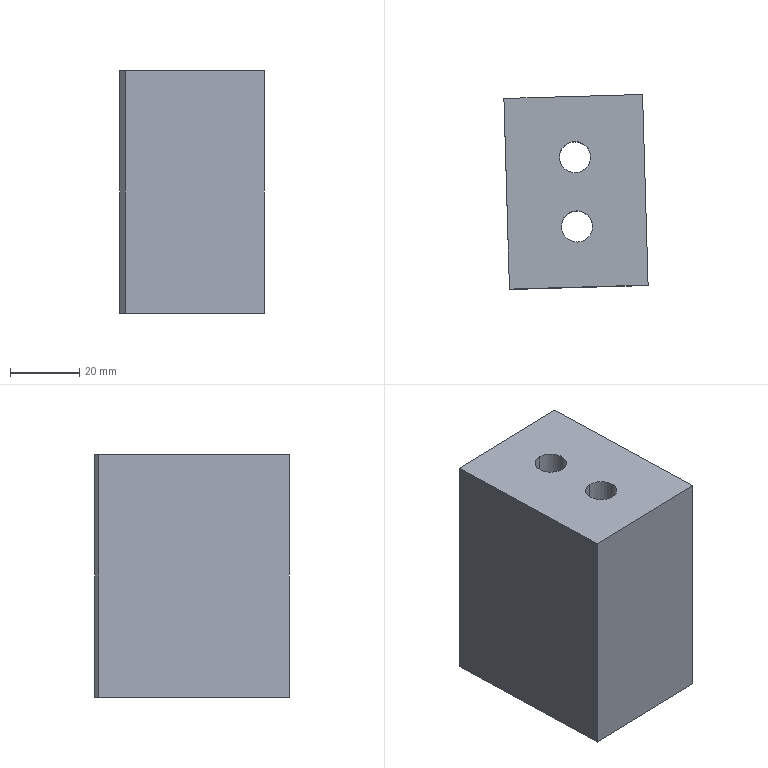Component | SolidWorks | NylonBlock6-1 | 1 solid | 16 faces | box 41.59 x 56.14 x 70 mm | volume 143148 mm3 | cylinder 8 | plane 8 | commonest cylinder face diameters 15 x4 9 x4 | material Nylon 101
build123d program:
from build123d import *

# Parameters (mm, degrees)
SKETCH1_W                                       = 55
SKETCH1_H                                       = 40
BOSS_EXTRUDE1_DEPTH                             = 35
M8_HEX_SOCKET_HEAD_CAP_SCREW_CBORE1_D           = 9
M8_HEX_SOCKET_HEAD_CAP_SCREW_CBORE1_CBORE_D     = 15
M8_HEX_SOCKET_HEAD_CAP_SCREW_CBORE1_CBORE_DEPTH = 8.6


with BuildPart() as part:
    # Sketch1 → Boss-Extrude1 (new, symmetric)
    with BuildSketch(Plane.XY):
        Rectangle(SKETCH1_W, SKETCH1_H)
    extrude(amount=BOSS_EXTRUDE1_DEPTH, both=True)

    # M8 Hex Socket Head Cap Screw CBORE1 (through all)
    with Locations(Plane(origin=(10, 0, -35), x_dir=(-1, 0, 0), z_dir=(0, 0, -1))):
        with Locations((0, 0), (20, 0)):
            CounterBoreHole(M8_HEX_SOCKET_HEAD_CAP_SCREW_CBORE1_D / 2, M8_HEX_SOCKET_HEAD_CAP_SCREW_CBORE1_CBORE_D / 2, M8_HEX_SOCKET_HEAD_CAP_SCREW_CBORE1_CBORE_DEPTH)


solid = part.part

# Placed as in the assembly
solid = solid.moved(Location((-297.687, -220.739, -1261.21), (0, 0, 91.672)))
STEP:
#1=COLOUR_RGB('',0.7922,0.8196,0.9333);
#2=FILL_AREA_STYLE_COLOUR('',#1);
#3=FILL_AREA_STYLE('',(#2));
#4=SURFACE_STYLE_FILL_AREA(#3);
#5=SURFACE_SIDE_STYLE('',(#4));
#6=SURFACE_STYLE_USAGE(.BOTH.,#5);
#7=PRESENTATION_STYLE_ASSIGNMENT((#6));
#8=CARTESIAN_POINT('',(-11.7,-9.379,-50.693));
#9=VERTEX_POINT('',#8);
#10=CARTESIAN_POINT('',(-11.717,-8.789,-50.693));
#11=VERTEX_POINT('',#10);
#12=CARTESIAN_POINT('',(-11.708,-9.084,-50.693));
#13=DIRECTION('',(-0.,0.,-1.));
#14=DIRECTION('',(-0.02918,0.9996,0.));
#15=AXIS2_PLACEMENT_3D('',#12,#13,#14);
#16=CIRCLE('',#15,0.2953);
#17=EDGE_CURVE('',#9,#11,#16,.T.);
#18=ORIENTED_EDGE('',*,*,#17,.F.);
#19=CARTESIAN_POINT('',(-11.7,-9.379,-51.032));
#20=VERTEX_POINT('',#19);
#21=CARTESIAN_POINT('',(-11.7,-9.379,-51.032));
#22=DIRECTION('',(-0.,0.,-1.));
#23=VECTOR('',#22,39.37);
#24=LINE('',#21,#23);
#25=EDGE_CURVE('',#9,#20,#24,.T.);
#26=ORIENTED_EDGE('',*,*,#25,.T.);
#27=CARTESIAN_POINT('',(-11.717,-8.789,-51.032));
#28=VERTEX_POINT('',#27);
#29=CARTESIAN_POINT('',(-11.708,-9.084,-51.032));
#30=DIRECTION('',(-0.,0.,-1.));
#31=DIRECTION('',(-0.02918,0.9996,0.));
#32=AXIS2_PLACEMENT_3D('',#29,#30,#31);
#33=CIRCLE('',#32,0.2953);
#34=EDGE_CURVE('',#20,#28,#33,.T.);
#35=ORIENTED_EDGE('',*,*,#34,.T.);
#36=CARTESIAN_POINT('',(-11.717,-8.789,-51.032));
#37=DIRECTION('',(-0.,0.,-1.));
#38=VECTOR('',#37,39.37);
#39=LINE('',#36,#38);
#40=EDGE_CURVE('',#11,#28,#39,.T.);
#41=ORIENTED_EDGE('',*,*,#40,.F.);
#42=EDGE_LOOP('',(#18,#26,#35,#41));
#43=FACE_OUTER_BOUND('',#42,.T.);
#44=CARTESIAN_POINT('',(-11.708,-9.084,-51.032));
#45=DIRECTION('',(-0.,0.,-1.));
#46=DIRECTION('',(-0.02918,0.9996,0.));
#47=AXIS2_PLACEMENT_3D('',#44,#45,#46);
#48=CYLINDRICAL_SURFACE('',#47,0.2953);
#49=ADVANCED_FACE('',(#43),#48,.F.);
#50=CARTESIAN_POINT('',(-11.703,-9.261,-48.276));
#51=VERTEX_POINT('',#50);
#52=CARTESIAN_POINT('',(-11.714,-8.907,-48.276));
#53=VERTEX_POINT('',#52);
#54=CARTESIAN_POINT('',(-11.708,-9.084,-48.276));
#55=DIRECTION('',(-0.,0.,-1.));
#56=DIRECTION('',(-0.02918,0.9996,0.));
#57=AXIS2_PLACEMENT_3D('',#54,#55,#56);
#58=CIRCLE('',#57,0.1772);
#59=EDGE_CURVE('',#51,#53,#58,.T.);
#60=ORIENTED_EDGE('',*,*,#59,.F.);
#61=CARTESIAN_POINT('',(-11.703,-9.261,-50.693));
#62=VERTEX_POINT('',#61);
#63=CARTESIAN_POINT('',(-11.703,-9.261,-51.032));
#64=DIRECTION('',(-0.,0.,-1.));
#65=VECTOR('',#64,39.37);
#66=LINE('',#63,#65);
#67=EDGE_CURVE('',#51,#62,#66,.T.);
#68=ORIENTED_EDGE('',*,*,#67,.T.);
#69=CARTESIAN_POINT('',(-11.714,-8.907,-50.693));
#70=VERTEX_POINT('',#69);
#71=CARTESIAN_POINT('',(-11.708,-9.084,-50.693));
#72=DIRECTION('',(-0.,0.,-1.));
#73=DIRECTION('',(-0.02918,0.9996,0.));
#74=AXIS2_PLACEMENT_3D('',#71,#72,#73);
#75=CIRCLE('',#74,0.1772);
#76=EDGE_CURVE('',#62,#70,#75,.T.);
#77=ORIENTED_EDGE('',*,*,#76,.T.);
#78=CARTESIAN_POINT('',(-11.714,-8.907,-51.032));
#79=DIRECTION('',(-0.,0.,-1.));
#80=VECTOR('',#79,39.37);
#81=LINE('',#78,#80);
#82=EDGE_CURVE('',#53,#70,#81,.T.);
#83=ORIENTED_EDGE('',*,*,#82,.F.);
#84=EDGE_LOOP('',(#60,#68,#77,#83));
#85=FACE_OUTER_BOUND('',#84,.T.);
#86=CARTESIAN_POINT('',(-11.708,-9.084,-51.032));
#87=DIRECTION('',(-0.,0.,-1.));
#88=DIRECTION('',(-0.02918,0.9996,0.));
#89=AXIS2_PLACEMENT_3D('',#86,#87,#88);
#90=CYLINDRICAL_SURFACE('',#89,0.1772);
#91=ADVANCED_FACE('',(#85),#90,.F.);
#92=CARTESIAN_POINT('',(-11.723,-8.592,-50.693));
#93=VERTEX_POINT('',#92);
#94=CARTESIAN_POINT('',(-11.74,-8.002,-50.693));
#95=VERTEX_POINT('',#94);
#96=CARTESIAN_POINT('',(-11.731,-8.297,-50.693));
#97=DIRECTION('',(-0.,0.,-1.));
#98=DIRECTION('',(-0.02918,0.9996,0.));
#99=AXIS2_PLACEMENT_3D('',#96,#97,#98);
#100=CIRCLE('',#99,0.2953);
#101=EDGE_CURVE('',#93,#95,#100,.T.);
#102=ORIENTED_EDGE('',*,*,#101,.F.);
#103=CARTESIAN_POINT('',(-11.723,-8.592,-51.032));
#104=VERTEX_POINT('',#103);
#105=CARTESIAN_POINT('',(-11.723,-8.592,-51.032));
#106=DIRECTION('',(-0.,0.,-1.));
#107=VECTOR('',#106,39.37);
#108=LINE('',#105,#107);
#109=EDGE_CURVE('',#93,#104,#108,.T.);
#110=ORIENTED_EDGE('',*,*,#109,.T.);
#111=CARTESIAN_POINT('',(-11.74,-8.002,-51.032));
#112=VERTEX_POINT('',#111);
#113=CARTESIAN_POINT('',(-11.731,-8.297,-51.032));
#114=DIRECTION('',(-0.,0.,-1.));
#115=DIRECTION('',(-0.02918,0.9996,0.));
#116=AXIS2_PLACEMENT_3D('',#113,#114,#115);
#117=CIRCLE('',#116,0.2953);
#118=EDGE_CURVE('',#104,#112,#117,.T.);
#119=ORIENTED_EDGE('',*,*,#118,.T.);
#120=CARTESIAN_POINT('',(-11.74,-8.002,-51.032));
#121=DIRECTION('',(-0.,0.,-1.));
#122=VECTOR('',#121,39.37);
#123=LINE('',#120,#122);
#124=EDGE_CURVE('',#95,#112,#123,.T.);
#125=ORIENTED_EDGE('',*,*,#124,.F.);
#126=EDGE_LOOP('',(#102,#110,#119,#125));
#127=FACE_OUTER_BOUND('',#126,.T.);
#128=CARTESIAN_POINT('',(-11.731,-8.297,-51.032));
#129=DIRECTION('',(-0.,0.,-1.));
#130=DIRECTION('',(-0.02918,0.9996,0.));
#131=AXIS2_PLACEMENT_3D('',#128,#129,#130);
#132=CYLINDRICAL_SURFACE('',#131,0.2953);
#133=ADVANCED_FACE('',(#127),#132,.F.);
#134=CARTESIAN_POINT('',(-11.726,-8.474,-48.276));
#135=VERTEX_POINT('',#134);
#136=CARTESIAN_POINT('',(-11.737,-8.12,-48.276));
#137=VERTEX_POINT('',#136);
#138=CARTESIAN_POINT('',(-11.731,-8.297,-48.276));
#139=DIRECTION('',(-0.,0.,-1.));
#140=DIRECTION('',(-0.02918,0.9996,0.));
#141=AXIS2_PLACEMENT_3D('',#138,#139,#140);
#142=CIRCLE('',#141,0.1772);
#143=EDGE_CURVE('',#135,#137,#142,.T.);
#144=ORIENTED_EDGE('',*,*,#143,.F.);
#145=CARTESIAN_POINT('',(-11.726,-8.474,-50.693));
#146=VERTEX_POINT('',#145);
#147=CARTESIAN_POINT('',(-11.726,-8.474,-51.032));
#148=DIRECTION('',(-0.,0.,-1.));
#149=VECTOR('',#148,39.37);
#150=LINE('',#147,#149);
#151=EDGE_CURVE('',#135,#146,#150,.T.);
#152=ORIENTED_EDGE('',*,*,#151,.T.);
#153=CARTESIAN_POINT('',(-11.737,-8.12,-50.693));
#154=VERTEX_POINT('',#153);
#155=CARTESIAN_POINT('',(-11.731,-8.297,-50.693));
#156=DIRECTION('',(-0.,0.,-1.));
#157=DIRECTION('',(-0.02918,0.9996,0.));
#158=AXIS2_PLACEMENT_3D('',#155,#156,#157);
#159=CIRCLE('',#158,0.1772);
#160=EDGE_CURVE('',#146,#154,#159,.T.);
#161=ORIENTED_EDGE('',*,*,#160,.T.);
#162=CARTESIAN_POINT('',(-11.737,-8.12,-51.032));
#163=DIRECTION('',(-0.,0.,-1.));
#164=VECTOR('',#163,39.37);
#165=LINE('',#162,#164);
#166=EDGE_CURVE('',#137,#154,#165,.T.);
#167=ORIENTED_EDGE('',*,*,#166,.F.);
#168=EDGE_LOOP('',(#144,#152,#161,#167));
#169=FACE_OUTER_BOUND('',#168,.T.);
#170=CARTESIAN_POINT('',(-11.731,-8.297,-51.032));
#171=DIRECTION('',(-0.,0.,-1.));
#172=DIRECTION('',(-0.02918,0.9996,0.));
#173=AXIS2_PLACEMENT_3D('',#170,#171,#172);
#174=CYLINDRICAL_SURFACE('',#173,0.1772);
#175=ADVANCED_FACE('',(#169),#174,.F.);
#176=CARTESIAN_POINT('',(-12.475,-9.796,-51.032));
#177=VERTEX_POINT('',#176);
#178=CARTESIAN_POINT('',(-10.901,-9.75,-51.032));
#179=VERTEX_POINT('',#178);
#180=CARTESIAN_POINT('',(-10.901,-9.75,-51.032));
#181=DIRECTION('',(0.9996,0.02918,-0.));
#182=VECTOR('',#181,39.37);
#183=LINE('',#180,#182);
#184=EDGE_CURVE('',#177,#179,#183,.T.);
#185=ORIENTED_EDGE('',*,*,#184,.T.);
#186=CARTESIAN_POINT('',(-10.901,-9.75,-48.276));
#187=VERTEX_POINT('',#186);
#188=CARTESIAN_POINT('',(-10.901,-9.75,-48.276));
#189=DIRECTION('',(-0.,0.,-1.));
#190=VECTOR('',#189,39.37);
#191=LINE('',#188,#190);
#192=EDGE_CURVE('',#187,#179,#191,.T.);
#193=ORIENTED_EDGE('',*,*,#192,.F.);
#194=CARTESIAN_POINT('',(-12.475,-9.796,-48.276));
#195=VERTEX_POINT('',#194);
#196=CARTESIAN_POINT('',(-10.901,-9.75,-48.276));
#197=DIRECTION('',(0.9996,0.02918,-0.));
#198=VECTOR('',#197,39.37);
#199=LINE('',#196,#198);
#200=EDGE_CURVE('',#195,#187,#199,.T.);
#201=ORIENTED_EDGE('',*,*,#200,.F.);
#202=CARTESIAN_POINT('',(-12.475,-9.796,-48.276));
#203=DIRECTION('',(-0.,0.,-1.));
#204=VECTOR('',#203,39.37);
#205=LINE('',#202,#204);
#206=EDGE_CURVE('',#195,#177,#205,.T.);
#207=ORIENTED_EDGE('',*,*,#206,.T.);
#208=EDGE_LOOP('',(#185,#193,#201,#207));
#209=FACE_OUTER_BOUND('',#208,.T.);
#210=CARTESIAN_POINT('',(-10.901,-9.75,-48.276));
#211=DIRECTION('',(-0.02918,0.9996,0.));
#212=DIRECTION('',(-0.9996,-0.02918,0.));
#213=AXIS2_PLACEMENT_3D('',#210,#211,#212);
#214=PLANE('',#213);
#215=ADVANCED_FACE('',(#209),#214,.F.);
#216=CARTESIAN_POINT('',(-10.964,-7.585,-51.032));
#217=VERTEX_POINT('',#216);
#218=CARTESIAN_POINT('',(-10.964,-7.585,-51.032));
#219=DIRECTION('',(-0.02918,0.9996,0.));
#220=VECTOR('',#219,39.37);
#221=LINE('',#218,#220);
#222=EDGE_CURVE('',#179,#217,#221,.T.);
#223=ORIENTED_EDGE('',*,*,#222,.T.);
#224=CARTESIAN_POINT('',(-10.964,-7.585,-48.276));
#225=VERTEX_POINT('',#224);
#226=CARTESIAN_POINT('',(-10.964,-7.585,-48.276));
#227=DIRECTION('',(-0.,0.,-1.));
#228=VECTOR('',#227,39.37);
#229=LINE('',#226,#228);
#230=EDGE_CURVE('',#225,#217,#229,.T.);
#231=ORIENTED_EDGE('',*,*,#230,.F.);
#232=CARTESIAN_POINT('',(-10.964,-7.585,-48.276));
#233=DIRECTION('',(-0.02918,0.9996,0.));
#234=VECTOR('',#233,39.37);
#235=LINE('',#232,#234);
#236=EDGE_CURVE('',#187,#225,#235,.T.);
#237=ORIENTED_EDGE('',*,*,#236,.F.);
#238=ORIENTED_EDGE('',*,*,#192,.T.);
#239=EDGE_LOOP('',(#223,#231,#237,#238));
#240=FACE_OUTER_BOUND('',#239,.T.);
#241=CARTESIAN_POINT('',(-10.964,-7.585,-48.276));
#242=DIRECTION('',(-0.9996,-0.02918,0.));
#243=DIRECTION('',(-0.,0.,-1.));
#244=AXIS2_PLACEMENT_3D('',#241,#242,#243);
#245=PLANE('',#244);
#246=ADVANCED_FACE('',(#240),#245,.F.);
#247=CARTESIAN_POINT('',(-12.539,-7.631,-51.032));
#248=VERTEX_POINT('',#247);
#249=CARTESIAN_POINT('',(-10.964,-7.585,-51.032));
#250=DIRECTION('',(-0.9996,-0.02918,0.));
#251=VECTOR('',#250,39.37);
#252=LINE('',#249,#251);
#253=EDGE_CURVE('',#217,#248,#252,.T.);
#254=ORIENTED_EDGE('',*,*,#253,.T.);
#255=CARTESIAN_POINT('',(-12.539,-7.631,-48.276));
#256=VERTEX_POINT('',#255);
#257=CARTESIAN_POINT('',(-12.539,-7.631,-48.276));
#258=DIRECTION('',(-0.,0.,-1.));
#259=VECTOR('',#258,39.37);
#260=LINE('',#257,#259);
#261=EDGE_CURVE('',#256,#248,#260,.T.);
#262=ORIENTED_EDGE('',*,*,#261,.F.);
#263=CARTESIAN_POINT('',(-10.964,-7.585,-48.276));
#264=DIRECTION('',(-0.9996,-0.02918,0.));
#265=VECTOR('',#264,39.37);
#266=LINE('',#263,#265);
#267=EDGE_CURVE('',#225,#256,#266,.T.);
#268=ORIENTED_EDGE('',*,*,#267,.F.);
#269=ORIENTED_EDGE('',*,*,#230,.T.);
#270=EDGE_LOOP('',(#254,#262,#268,#269));
#271=FACE_OUTER_BOUND('',#270,.T.);
#272=CARTESIAN_POINT('',(-10.964,-7.585,-48.276));
#273=DIRECTION('',(0.02918,-0.9996,-0.));
#274=DIRECTION('',(0.9996,0.02918,-0.));
#275=AXIS2_PLACEMENT_3D('',#272,#273,#274);
#276=PLANE('',#275);
#277=ADVANCED_FACE('',(#271),#276,.F.);
#278=CARTESIAN_POINT('',(-12.539,-7.631,-51.032));
#279=DIRECTION('',(0.02918,-0.9996,-0.));
#280=VECTOR('',#279,39.37);
#281=LINE('',#278,#280);
#282=EDGE_CURVE('',#248,#177,#281,.T.);
#283=ORIENTED_EDGE('',*,*,#282,.T.);
#284=ORIENTED_EDGE('',*,*,#206,.F.);
#285=CARTESIAN_POINT('',(-12.539,-7.631,-48.276));
#286=DIRECTION('',(0.02918,-0.9996,-0.));
#287=VECTOR('',#286,39.37);
#288=LINE('',#285,#287);
#289=EDGE_CURVE('',#256,#195,#288,.T.);
#290=ORIENTED_EDGE('',*,*,#289,.F.);
#291=ORIENTED_EDGE('',*,*,#261,.T.);
#292=EDGE_LOOP('',(#283,#284,#290,#291));
#293=FACE_OUTER_BOUND('',#292,.T.);
#294=CARTESIAN_POINT('',(-12.539,-7.631,-48.276));
#295=DIRECTION('',(0.9996,0.02918,-0.));
#296=DIRECTION('',(0.,-0.,1.));
#297=AXIS2_PLACEMENT_3D('',#294,#295,#296);
#298=PLANE('',#297);
#299=ADVANCED_FACE('',(#293),#298,.F.);
#300=CARTESIAN_POINT('',(-11.708,-9.084,-48.276));
#301=DIRECTION('',(-0.,0.,-1.));
#302=DIRECTION('',(-0.02918,0.9996,0.));
#303=AXIS2_PLACEMENT_3D('',#300,#301,#302);
#304=CIRCLE('',#303,0.1772);
#305=EDGE_CURVE('',#53,#51,#304,.T.);
#306=ORIENTED_EDGE('',*,*,#305,.T.);
#307=ORIENTED_EDGE('',*,*,#59,.T.);
#308=EDGE_LOOP('',(#306,#307));
#309=FACE_BOUND('',#308,.T.);
#310=CARTESIAN_POINT('',(-11.731,-8.297,-48.276));
#311=DIRECTION('',(-0.,0.,-1.));
#312=DIRECTION('',(-0.02918,0.9996,0.));
#313=AXIS2_PLACEMENT_3D('',#310,#311,#312);
#314=CIRCLE('',#313,0.1772);
#315=EDGE_CURVE('',#137,#135,#314,.T.);
#316=ORIENTED_EDGE('',*,*,#315,.T.);
#317=ORIENTED_EDGE('',*,*,#143,.T.);
#318=EDGE_LOOP('',(#316,#317));
#319=FACE_BOUND('',#318,.T.);
#320=ORIENTED_EDGE('',*,*,#200,.T.);
#321=ORIENTED_EDGE('',*,*,#236,.T.);
#322=ORIENTED_EDGE('',*,*,#267,.T.);
#323=ORIENTED_EDGE('',*,*,#289,.T.);
#324=EDGE_LOOP('',(#320,#321,#322,#323));
#325=FACE_OUTER_BOUND('',#324,.T.);
#326=CARTESIAN_POINT('',(-11.72,-8.691,-48.276));
#327=DIRECTION('',(0.,-0.,1.));
#328=DIRECTION('',(0.02918,-0.9996,-0.));
#329=AXIS2_PLACEMENT_3D('',#326,#327,#328);
#330=PLANE('',#329);
#331=ADVANCED_FACE('',(#309,#319,#325),#330,.T.);
#332=CARTESIAN_POINT('',(-11.708,-9.084,-51.032));
#333=DIRECTION('',(-0.,0.,-1.));
#334=DIRECTION('',(-0.02918,0.9996,0.));
#335=AXIS2_PLACEMENT_3D('',#332,#333,#334);
#336=CIRCLE('',#335,0.2953);
#337=EDGE_CURVE('',#28,#20,#336,.T.);
#338=ORIENTED_EDGE('',*,*,#337,.F.);
#339=ORIENTED_EDGE('',*,*,#34,.F.);
#340=EDGE_LOOP('',(#338,#339));
#341=FACE_BOUND('',#340,.T.);
#342=CARTESIAN_POINT('',(-11.731,-8.297,-51.032));
#343=DIRECTION('',(-0.,0.,-1.));
#344=DIRECTION('',(-0.02918,0.9996,0.));
#345=AXIS2_PLACEMENT_3D('',#342,#343,#344);
#346=CIRCLE('',#345,0.2953);
#347=EDGE_CURVE('',#112,#104,#346,.T.);
#348=ORIENTED_EDGE('',*,*,#347,.F.);
#349=ORIENTED_EDGE('',*,*,#118,.F.);
#350=EDGE_LOOP('',(#348,#349));
#351=FACE_BOUND('',#350,.T.);
#352=ORIENTED_EDGE('',*,*,#184,.F.);
#353=ORIENTED_EDGE('',*,*,#282,.F.);
#354=ORIENTED_EDGE('',*,*,#253,.F.);
#355=ORIENTED_EDGE('',*,*,#222,.F.);
#356=EDGE_LOOP('',(#352,#353,#354,#355));
#357=FACE_OUTER_BOUND('',#356,.T.);
#358=CARTESIAN_POINT('',(-11.72,-8.691,-51.032));
#359=DIRECTION('',(0.,-0.,1.));
#360=DIRECTION('',(0.02918,-0.9996,-0.));
#361=AXIS2_PLACEMENT_3D('',#358,#359,#360);
#362=PLANE('',#361);
#363=ADVANCED_FACE('',(#341,#351,#357),#362,.F.);
#364=ORIENTED_EDGE('',*,*,#151,.F.);
#365=ORIENTED_EDGE('',*,*,#315,.F.);
#366=ORIENTED_EDGE('',*,*,#166,.T.);
#367=CARTESIAN_POINT('',(-11.731,-8.297,-50.693));
#368=DIRECTION('',(-0.,0.,-1.));
#369=DIRECTION('',(-0.02918,0.9996,0.));
#370=AXIS2_PLACEMENT_3D('',#367,#368,#369);
#371=CIRCLE('',#370,0.1772);
#372=EDGE_CURVE('',#154,#146,#371,.T.);
#373=ORIENTED_EDGE('',*,*,#372,.T.);
#374=EDGE_LOOP('',(#364,#365,#366,#373));
#375=FACE_OUTER_BOUND('',#374,.T.);
#376=CARTESIAN_POINT('',(-11.731,-8.297,-51.032));
#377=DIRECTION('',(-0.,0.,-1.));
#378=DIRECTION('',(-0.02918,0.9996,0.));
#379=AXIS2_PLACEMENT_3D('',#376,#377,#378);
#380=CYLINDRICAL_SURFACE('',#379,0.1772);
#381=ADVANCED_FACE('',(#375),#380,.F.);
#382=ORIENTED_EDGE('',*,*,#372,.F.);
#383=ORIENTED_EDGE('',*,*,#160,.F.);
#384=EDGE_LOOP('',(#382,#383));
#385=FACE_BOUND('',#384,.T.);
#386=CARTESIAN_POINT('',(-11.731,-8.297,-50.693));
#387=DIRECTION('',(-0.,0.,-1.));
#388=DIRECTION('',(-0.02918,0.9996,0.));
#389=AXIS2_PLACEMENT_3D('',#386,#387,#388);
#390=CIRCLE('',#389,0.2953);
#391=EDGE_CURVE('',#95,#93,#390,.T.);
#392=ORIENTED_EDGE('',*,*,#391,.T.);
#393=ORIENTED_EDGE('',*,*,#101,.T.);
#394=EDGE_LOOP('',(#392,#393));
#395=FACE_OUTER_BOUND('',#394,.T.);
#396=CARTESIAN_POINT('',(-11.726,-8.474,-50.693));
#397=DIRECTION('',(0.,-0.,1.));
#398=DIRECTION('',(0.02918,-0.9996,-0.));
#399=AXIS2_PLACEMENT_3D('',#396,#397,#398);
#400=PLANE('',#399);
#401=ADVANCED_FACE('',(#385,#395),#400,.F.);
#402=ORIENTED_EDGE('',*,*,#109,.F.);
#403=ORIENTED_EDGE('',*,*,#391,.F.);
#404=ORIENTED_EDGE('',*,*,#124,.T.);
#405=ORIENTED_EDGE('',*,*,#347,.T.);
#406=EDGE_LOOP('',(#402,#403,#404,#405));
#407=FACE_OUTER_BOUND('',#406,.T.);
#408=CARTESIAN_POINT('',(-11.731,-8.297,-51.032));
#409=DIRECTION('',(-0.,0.,-1.));
#410=DIRECTION('',(-0.02918,0.9996,0.));
#411=AXIS2_PLACEMENT_3D('',#408,#409,#410);
#412=CYLINDRICAL_SURFACE('',#411,0.2953);
#413=ADVANCED_FACE('',(#407),#412,.F.);
#414=ORIENTED_EDGE('',*,*,#67,.F.);
#415=ORIENTED_EDGE('',*,*,#305,.F.);
#416=ORIENTED_EDGE('',*,*,#82,.T.);
#417=CARTESIAN_POINT('',(-11.708,-9.084,-50.693));
#418=DIRECTION('',(-0.,0.,-1.));
#419=DIRECTION('',(-0.02918,0.9996,0.));
#420=AXIS2_PLACEMENT_3D('',#417,#418,#419);
#421=CIRCLE('',#420,0.1772);
#422=EDGE_CURVE('',#70,#62,#421,.T.);
#423=ORIENTED_EDGE('',*,*,#422,.T.);
#424=EDGE_LOOP('',(#414,#415,#416,#423));
#425=FACE_OUTER_BOUND('',#424,.T.);
#426=CARTESIAN_POINT('',(-11.708,-9.084,-51.032));
#427=DIRECTION('',(-0.,0.,-1.));
#428=DIRECTION('',(-0.02918,0.9996,0.));
#429=AXIS2_PLACEMENT_3D('',#426,#427,#428);
#430=CYLINDRICAL_SURFACE('',#429,0.1772);
#431=ADVANCED_FACE('',(#425),#430,.F.);
#432=ORIENTED_EDGE('',*,*,#422,.F.);
#433=ORIENTED_EDGE('',*,*,#76,.F.);
#434=EDGE_LOOP('',(#432,#433));
#435=FACE_BOUND('',#434,.T.);
#436=CARTESIAN_POINT('',(-11.708,-9.084,-50.693));
#437=DIRECTION('',(-0.,0.,-1.));
#438=DIRECTION('',(-0.02918,0.9996,0.));
#439=AXIS2_PLACEMENT_3D('',#436,#437,#438);
#440=CIRCLE('',#439,0.2953);
#441=EDGE_CURVE('',#11,#9,#440,.T.);
#442=ORIENTED_EDGE('',*,*,#441,.T.);
#443=ORIENTED_EDGE('',*,*,#17,.T.);
#444=EDGE_LOOP('',(#442,#443));
#445=FACE_OUTER_BOUND('',#444,.T.);
#446=CARTESIAN_POINT('',(-11.703,-9.261,-50.693));
#447=DIRECTION('',(0.,-0.,1.));
#448=DIRECTION('',(0.02918,-0.9996,-0.));
#449=AXIS2_PLACEMENT_3D('',#446,#447,#448);
#450=PLANE('',#449);
#451=ADVANCED_FACE('',(#435,#445),#450,.F.);
#452=ORIENTED_EDGE('',*,*,#25,.F.);
#453=ORIENTED_EDGE('',*,*,#441,.F.);
#454=ORIENTED_EDGE('',*,*,#40,.T.);
#455=ORIENTED_EDGE('',*,*,#337,.T.);
#456=EDGE_LOOP('',(#452,#453,#454,#455));
#457=FACE_OUTER_BOUND('',#456,.T.);
#458=CARTESIAN_POINT('',(-11.708,-9.084,-51.032));
#459=DIRECTION('',(-0.,0.,-1.));
#460=DIRECTION('',(-0.02918,0.9996,0.));
#461=AXIS2_PLACEMENT_3D('',#458,#459,#460);
#462=CYLINDRICAL_SURFACE('',#461,0.2953);
#463=ADVANCED_FACE('',(#457),#462,.F.);
#464=CLOSED_SHELL('',(#49,#91,#133,#175,#215,#246,#277,#299,#331,#363,#381,#401,#413,#431,#451,#463));
#465=MANIFOLD_SOLID_BREP('',#464);
#466=STYLED_ITEM('',(#7),#465);
#467=PRESENTATION_LAYER_ASSIGNMENT('','',(#466));
#468=CARTESIAN_POINT('',(0.,0.,0.));
#469=DIRECTION('',(0.,0.,1.));
#470=DIRECTION('',(1.,0.,0.));
#471=AXIS2_PLACEMENT_3D('',#468,#469,#470);
#472=(LENGTH_UNIT()NAMED_UNIT(*)SI_UNIT($,.METRE.));
#473=LENGTH_MEASURE_WITH_UNIT(LENGTH_MEASURE(0.0254),#472);
#474=DIMENSIONAL_EXPONENTS(1.,0.,0.,0.,0.,0.,0.);
#475=(CONVERSION_BASED_UNIT('',#473)LENGTH_UNIT()NAMED_UNIT(#474));
#476=UNCERTAINTY_MEASURE_WITH_UNIT(LENGTH_MEASURE(0.00001),#475,'','');
#477=(NAMED_UNIT(*)PLANE_ANGLE_UNIT()SI_UNIT($,.RADIAN.));
#478=(NAMED_UNIT(*)SI_UNIT($,.STERADIAN.)SOLID_ANGLE_UNIT());
#479=(GEOMETRIC_REPRESENTATION_CONTEXT(3)GLOBAL_UNCERTAINTY_ASSIGNED_CONTEXT((#476))GLOBAL_UNIT_ASSIGNED_CONTEXT((#475,#477,#478))REPRESENTATION_CONTEXT('',''));
#480=ADVANCED_BREP_SHAPE_REPRESENTATION('',(#465,#471),#479);
#481=(LENGTH_UNIT()NAMED_UNIT(*)SI_UNIT($,.METRE.));
#482=LENGTH_MEASURE_WITH_UNIT(LENGTH_MEASURE(0.0254),#481);
#483=DIMENSIONAL_EXPONENTS(1.,0.,0.,0.,0.,0.,0.);
#484=(CONVERSION_BASED_UNIT('',#482)LENGTH_UNIT()NAMED_UNIT(#483));
#485=UNCERTAINTY_MEASURE_WITH_UNIT(LENGTH_MEASURE(0.00001),#484,'','');
#486=(NAMED_UNIT(*)PLANE_ANGLE_UNIT()SI_UNIT($,.RADIAN.));
#487=(NAMED_UNIT(*)SI_UNIT($,.STERADIAN.)SOLID_ANGLE_UNIT());
#488=(GEOMETRIC_REPRESENTATION_CONTEXT(3)GLOBAL_UNCERTAINTY_ASSIGNED_CONTEXT((#485))GLOBAL_UNIT_ASSIGNED_CONTEXT((#484,#486,#487))REPRESENTATION_CONTEXT('',''));
#489=MECHANICAL_DESIGN_GEOMETRIC_PRESENTATION_REPRESENTATION('',(#466),#488);